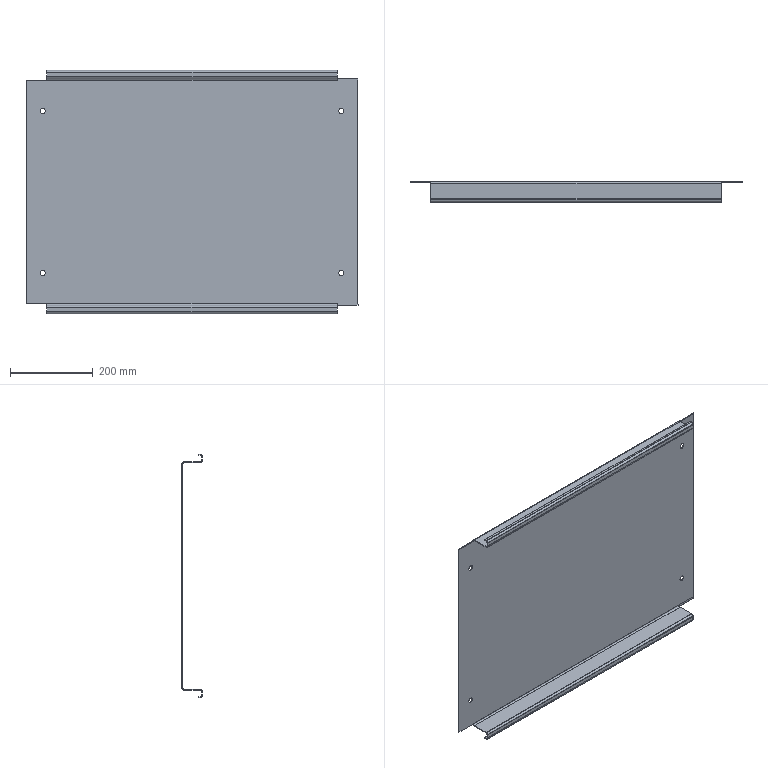Component | SolidWorks | UpperBaffle-1 | 1 solid | 66 faces | volume 1068367 mm3 | plane 46 | cylinder 20 | commonest cylinder face diameters 12.5 x8 11 x6 7 x6